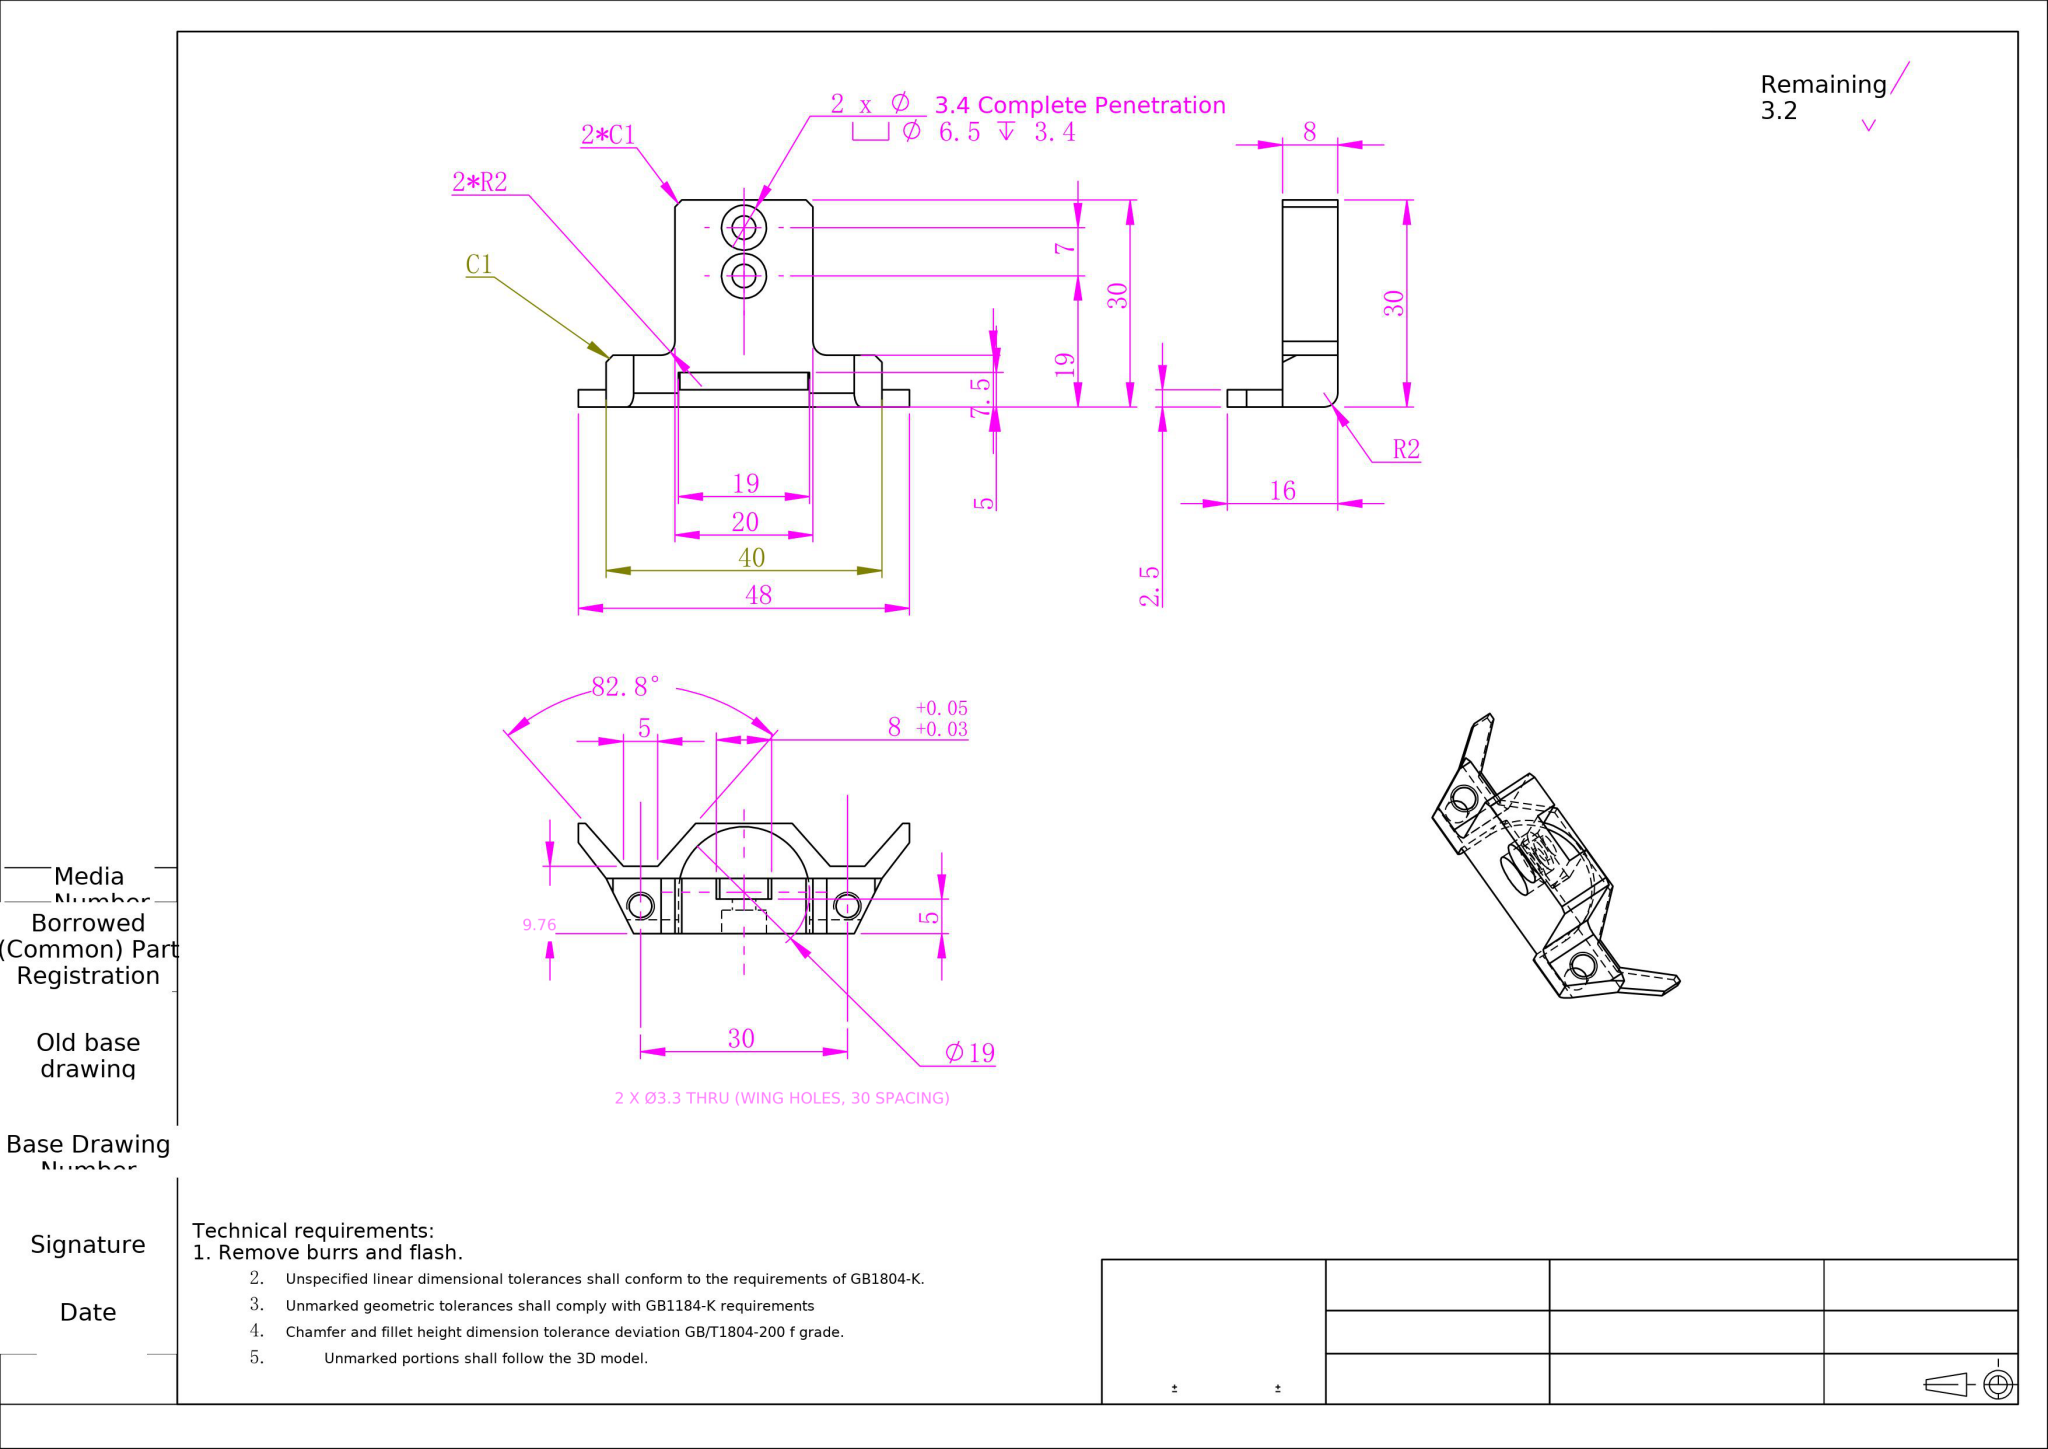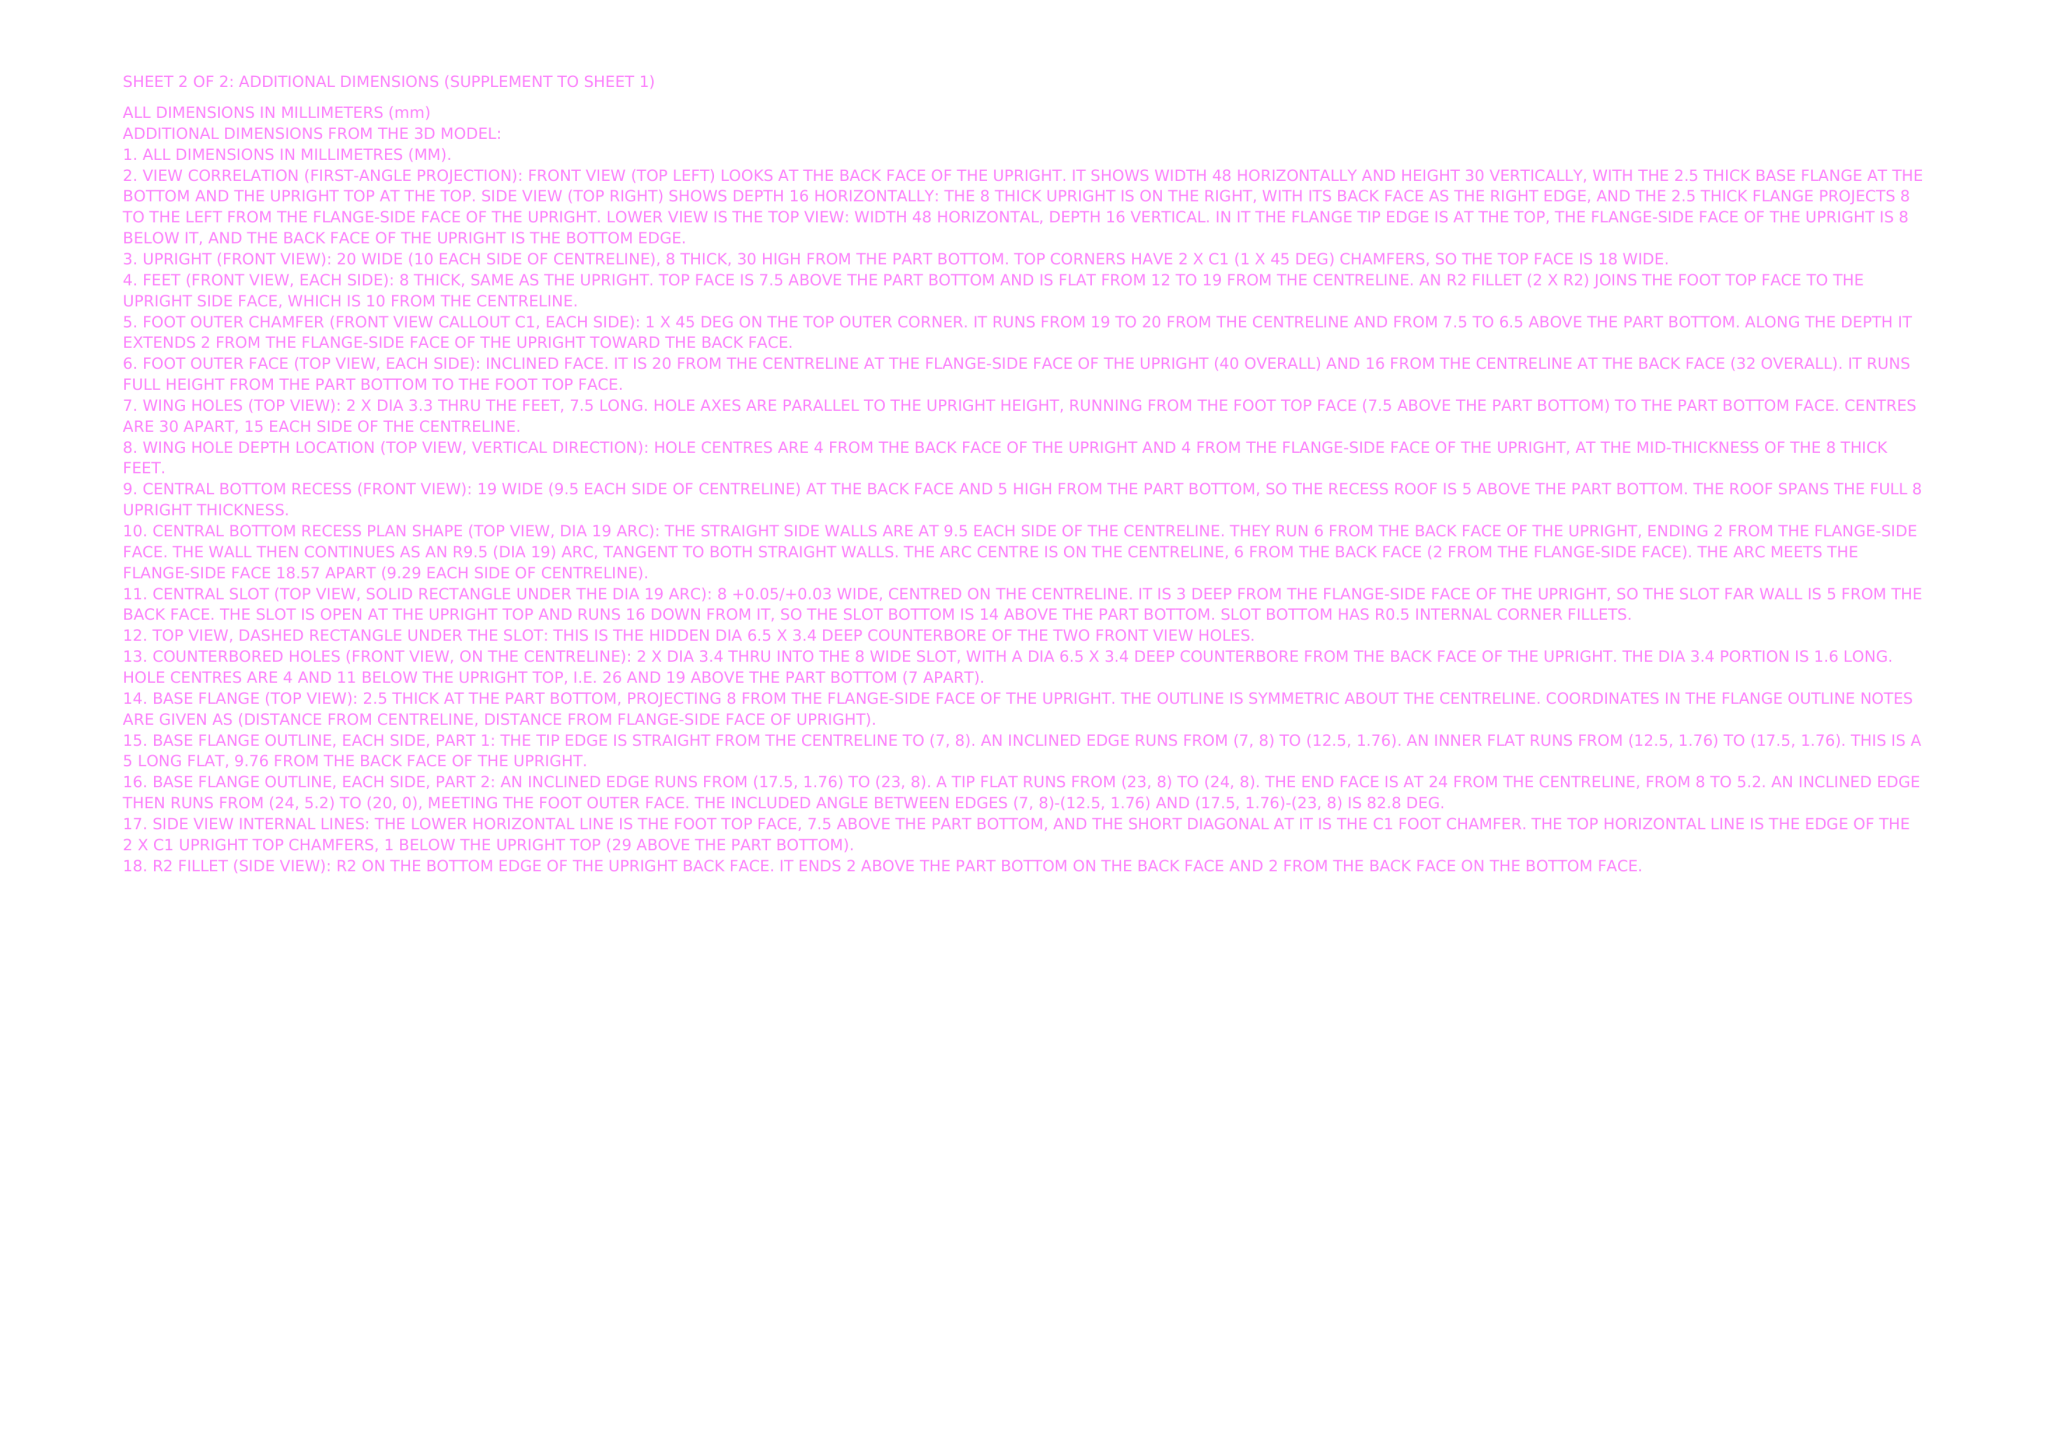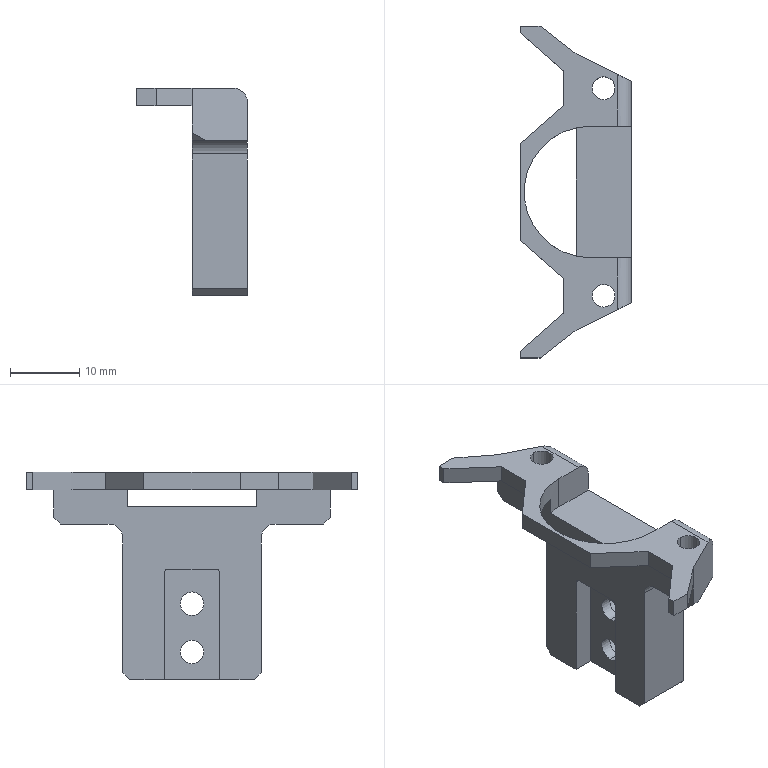Part | NX | mm | 1 solid | 56 faces | box 16 x 48 x 30 mm | volume 4549 mm3 | plane 37 | cylinder 19 | commonest cylinder face diameters 3.3 x4 6.5 x4 3.4 x4 4 x4 1 x2 19 x1